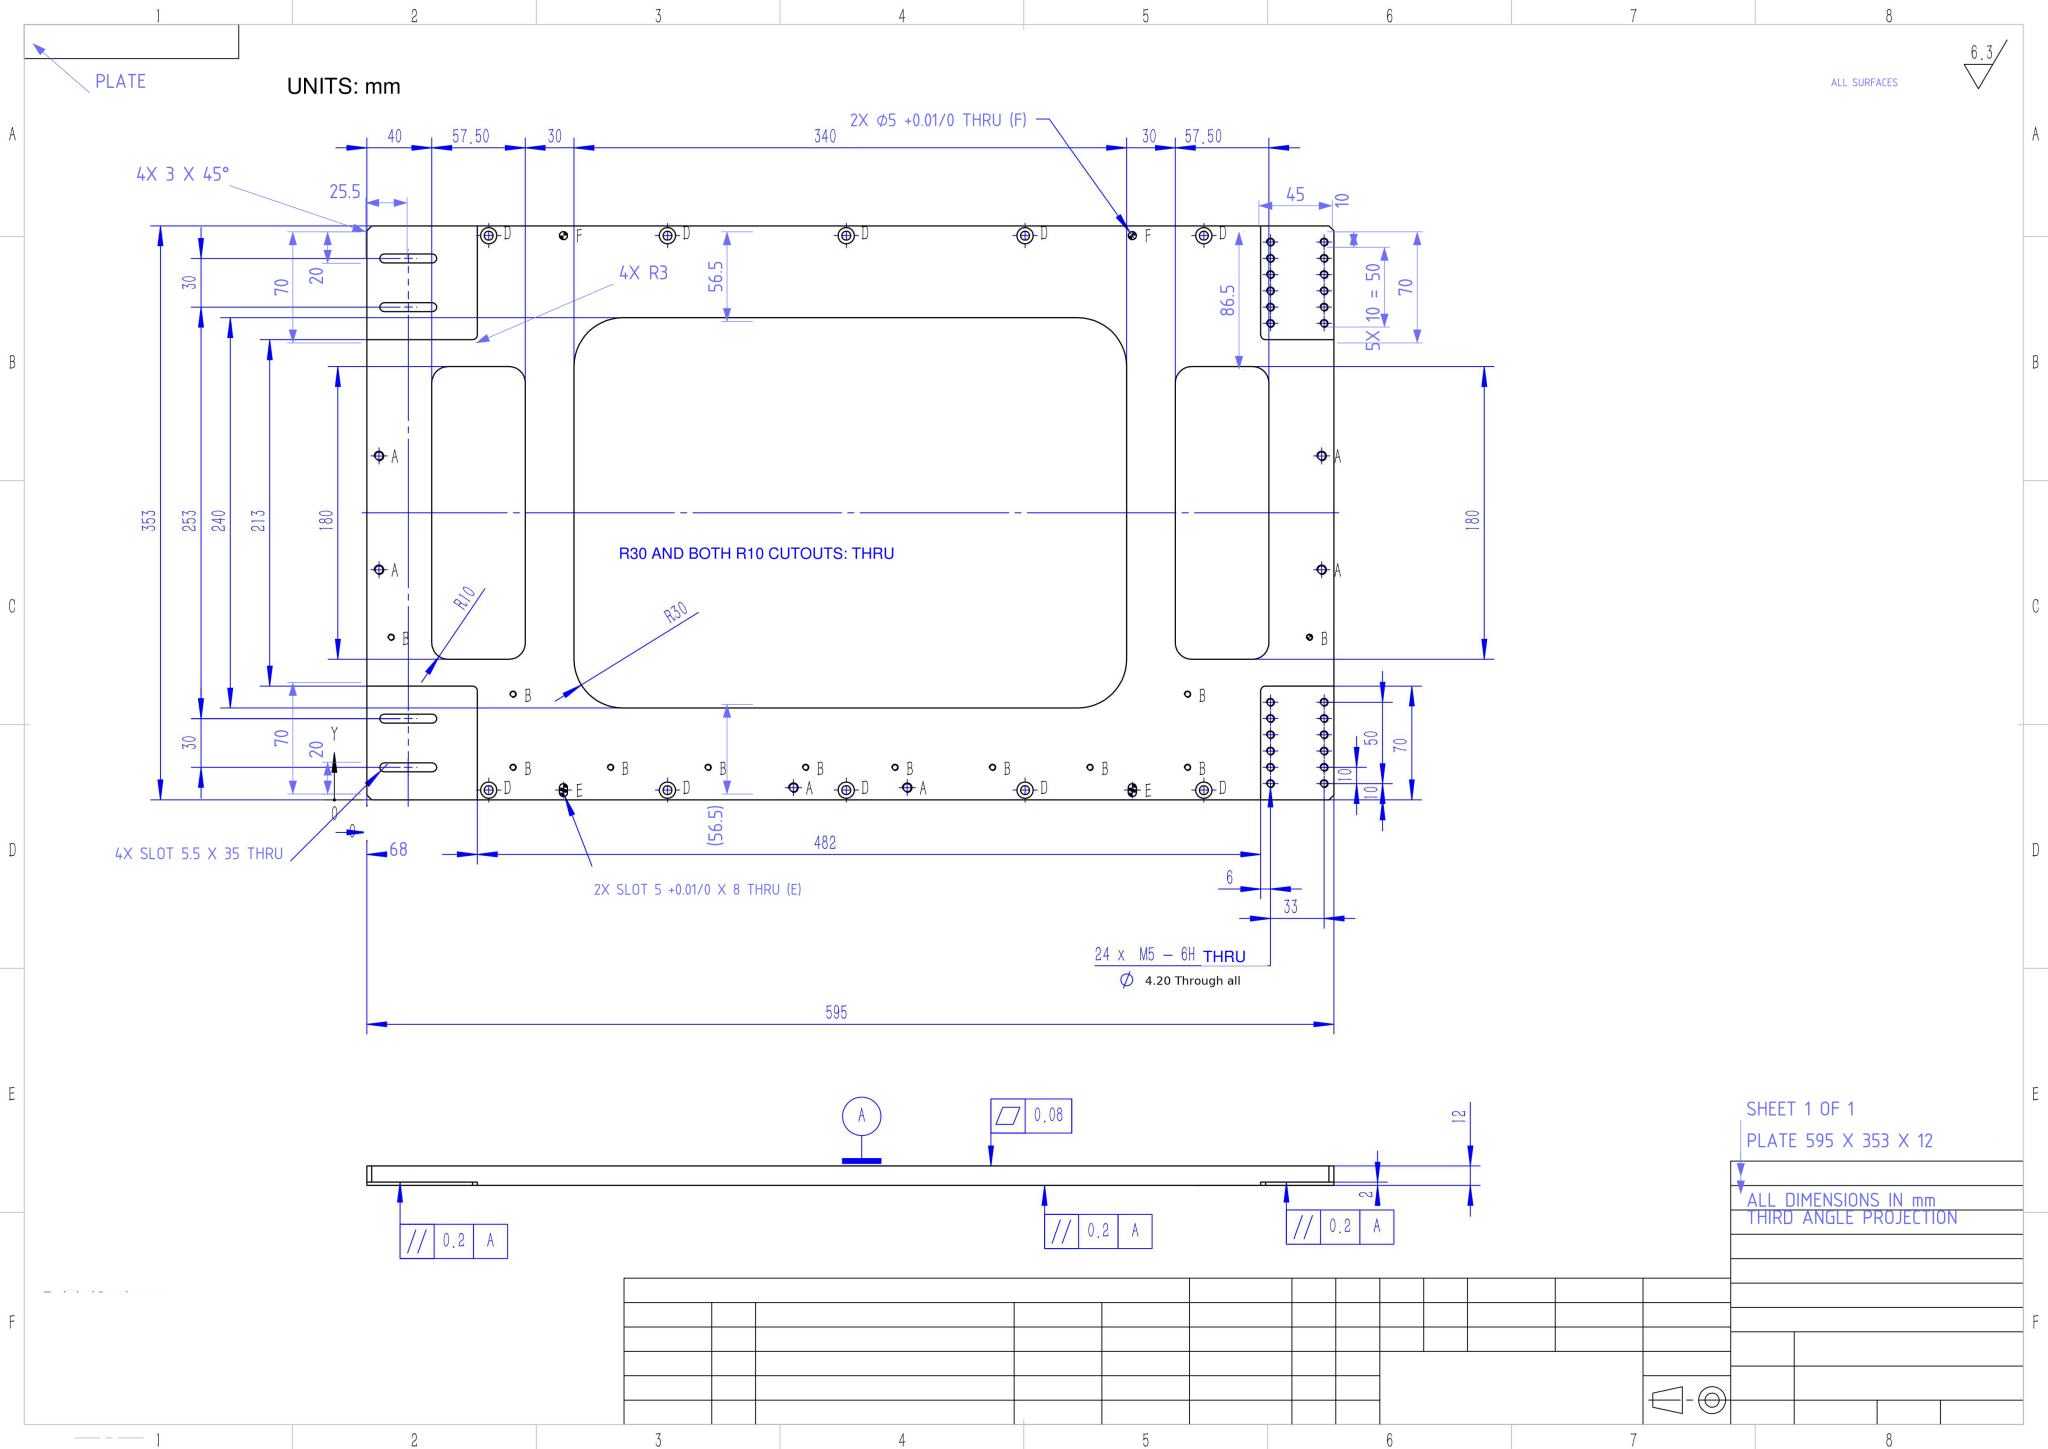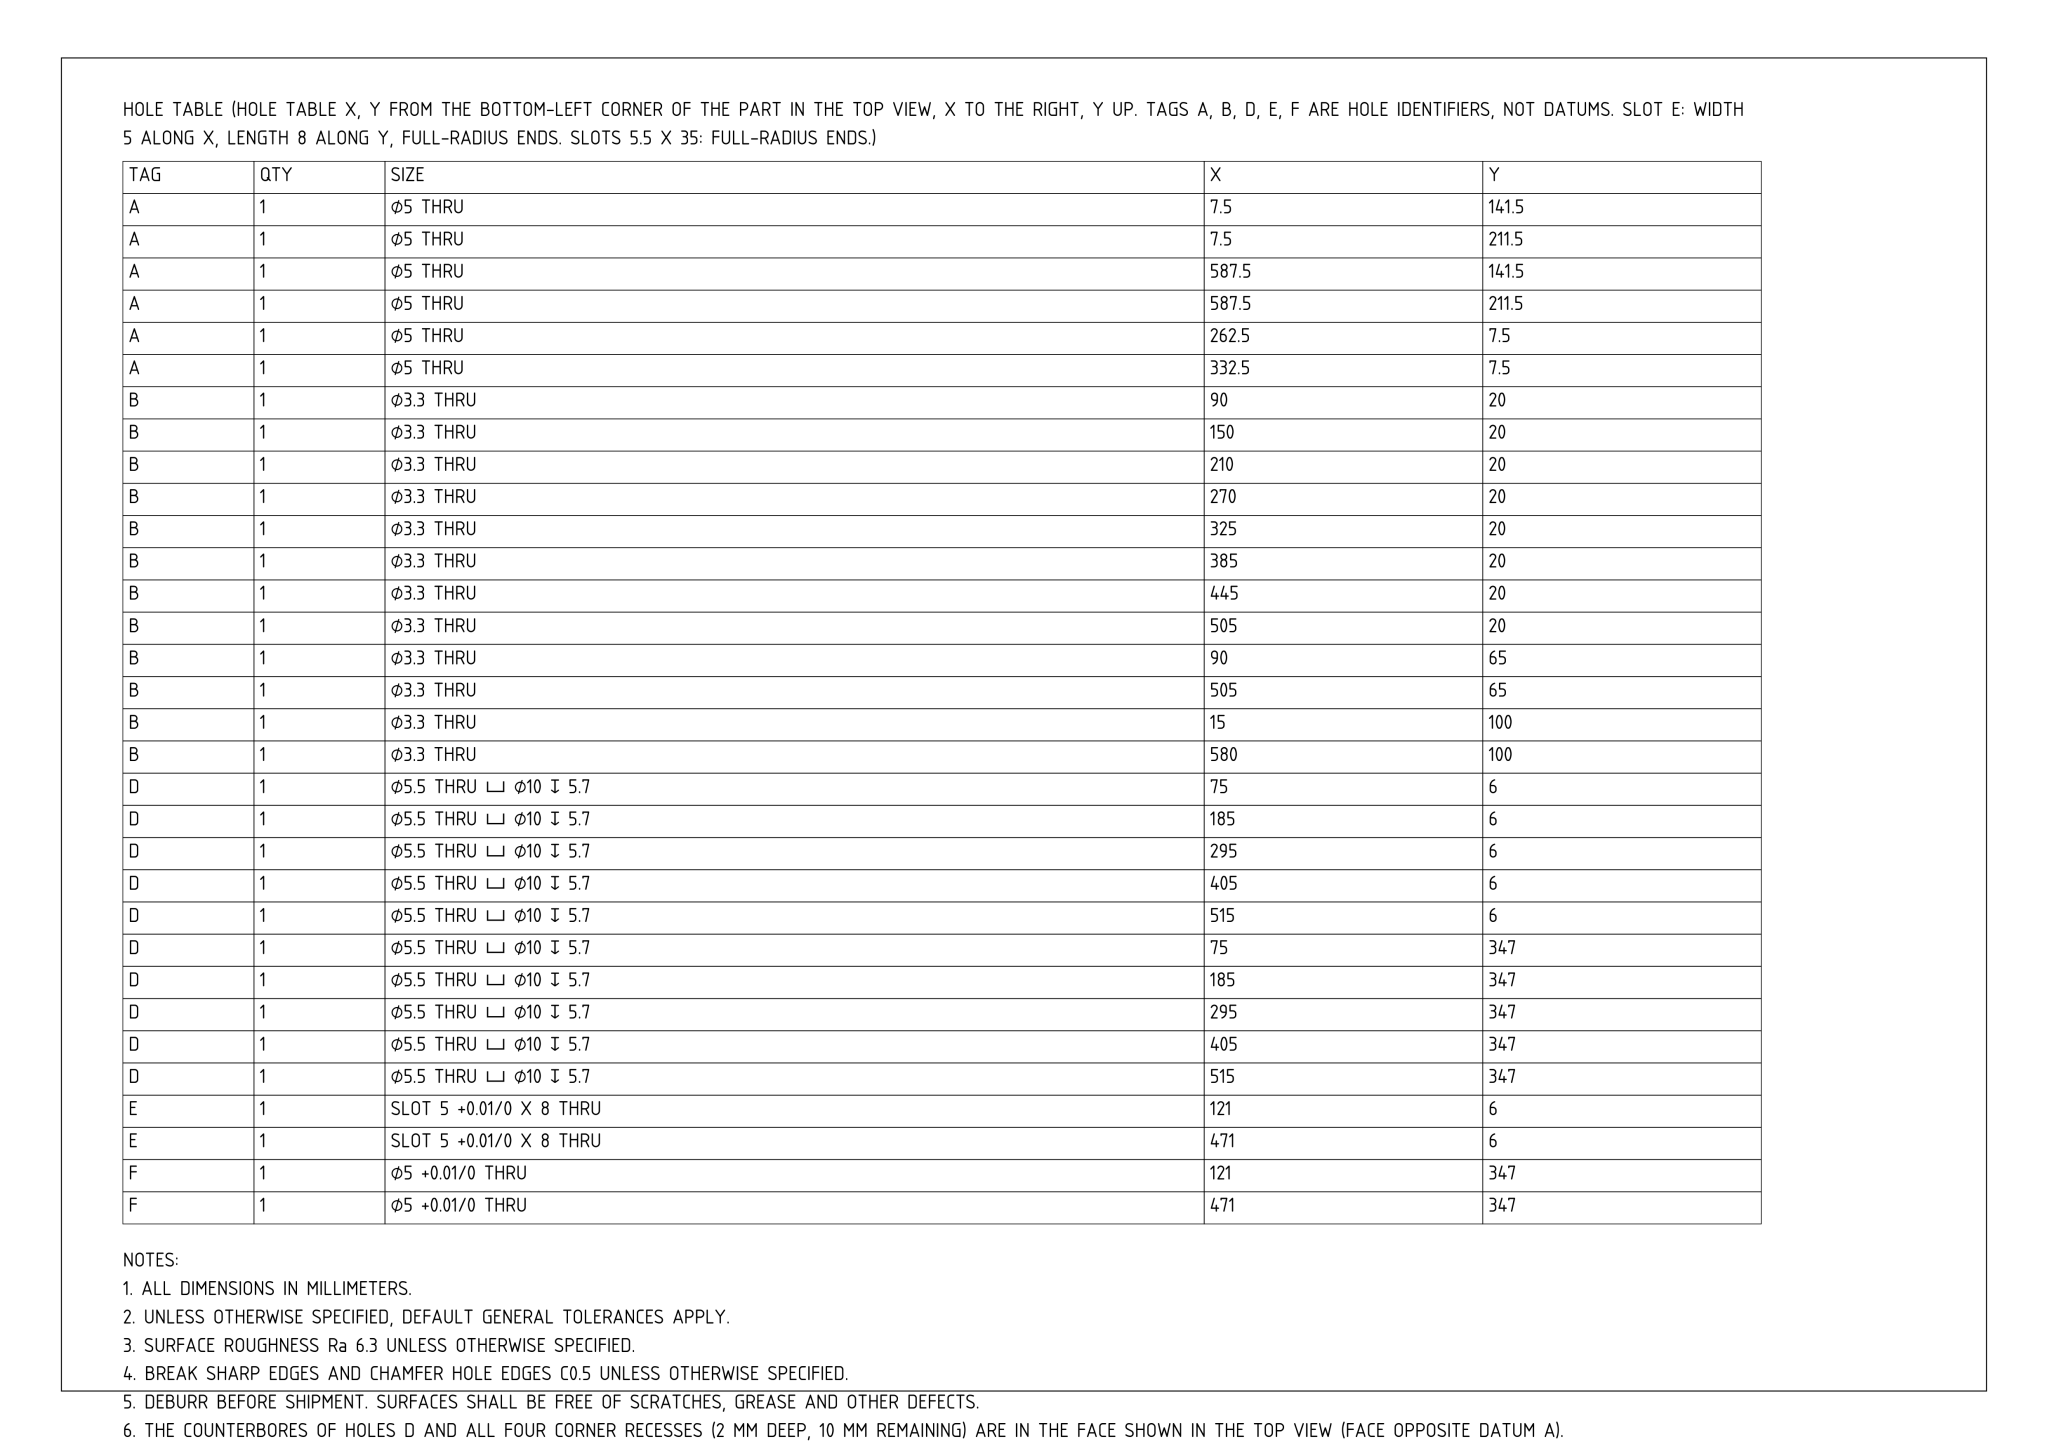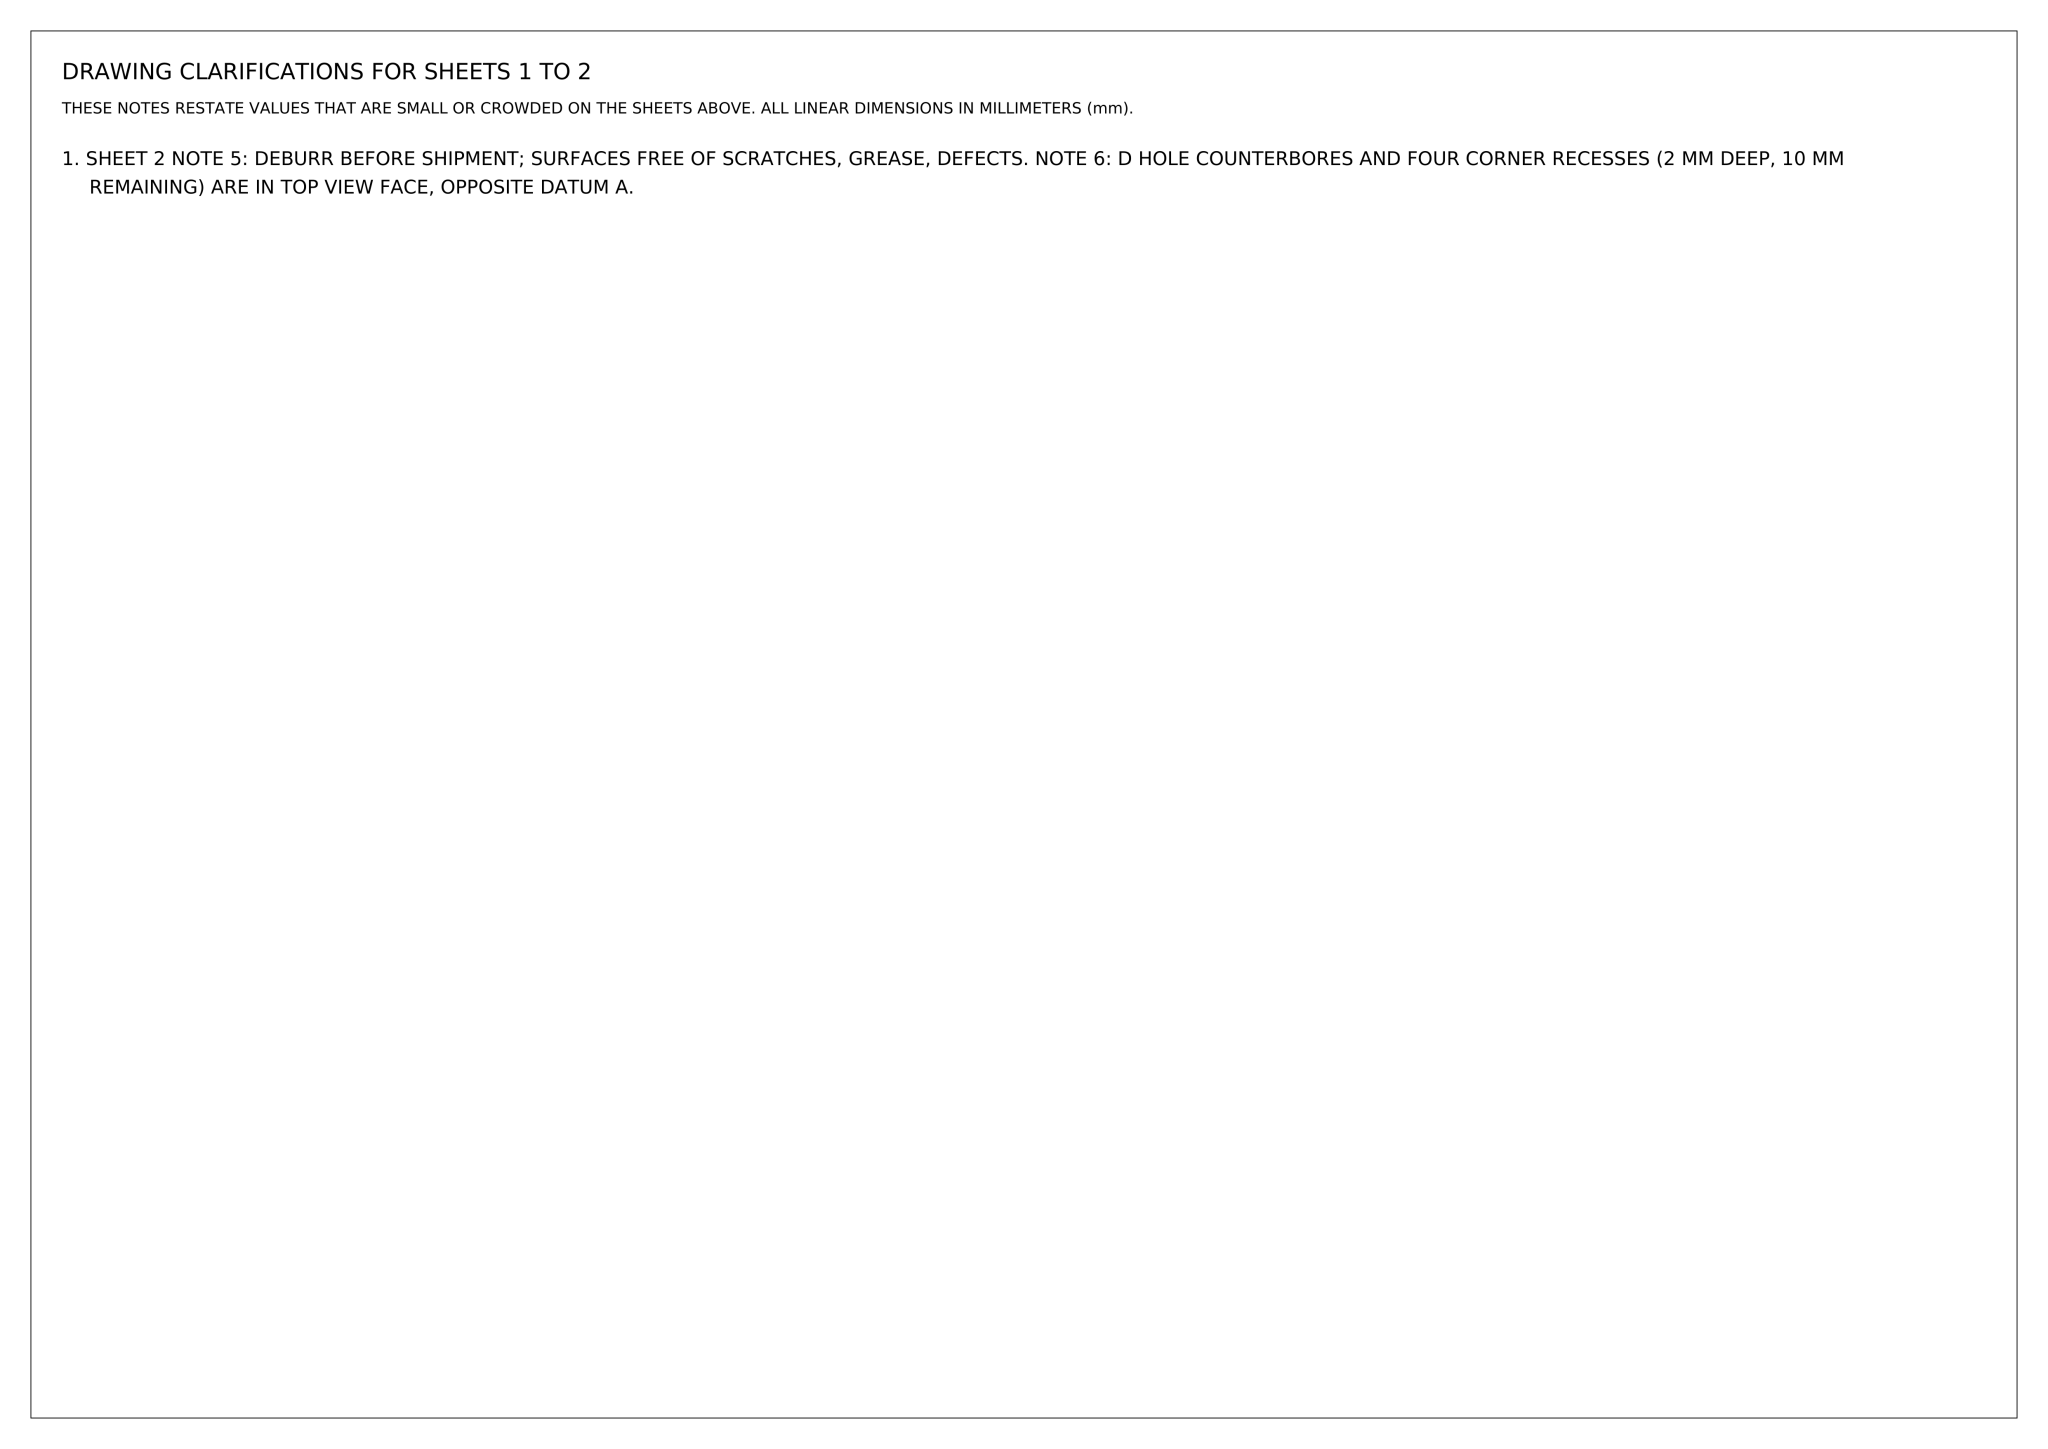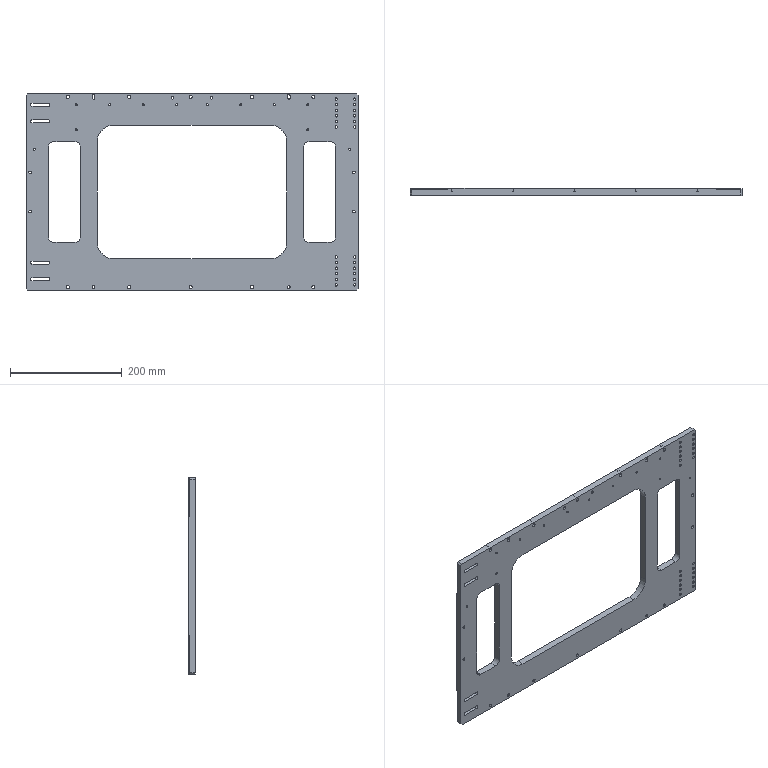Part | NX | mm | 1 solid | 214 faces | box 595 x 12 x 353 mm | volume 1251660 mm3 | cylinder 158 | plane 56 | commonest cylinder face diameters 4.2 x48 5.5 x28 3.3 x24 5 x22 10 x20 20 x8 60 x4 6 x4